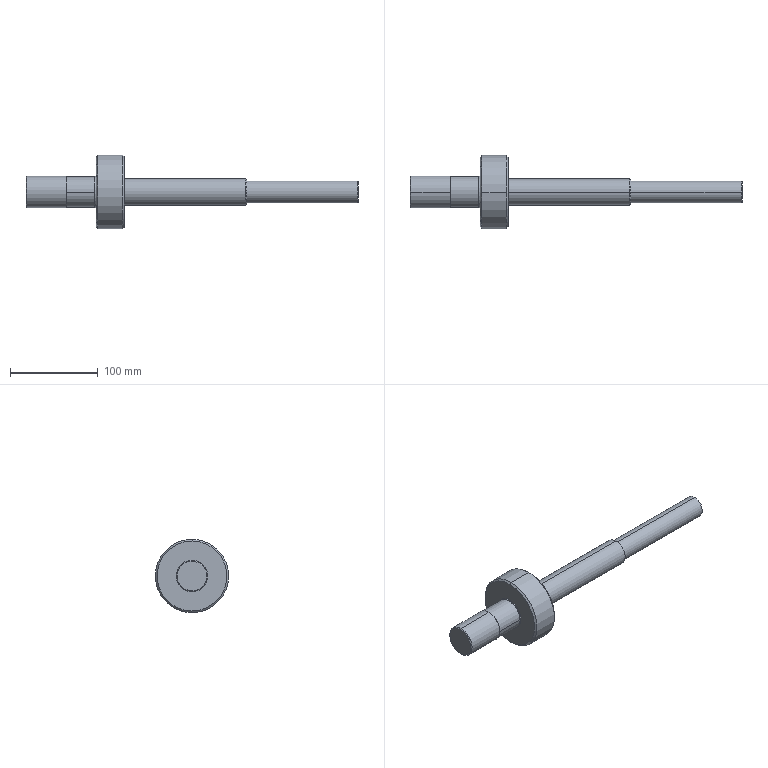Component | SolidWorks | 216InnerTubeAssembly-1_Mandrel1-1 | 1 solid | 29 faces | box 379 x 84 x 84 mm | volume 417048 mm3 | cylinder 12 | cone 10 | plane 7 | commonest cylinder face diameters 36 x4 34.99 x2 25 x2 30 x2 84 x2 | material Alloy Steel
build123d program:
from build123d import *

# Parameters (mm, degrees)
SKETCH1_W = 32.7
SKETCH1_H = 1.005


with BuildPart() as part:
    # Model → Revolve1 (revolve)
    with BuildSketch(Plane.XY, mode=Mode.PRIVATE) as revolve1_sk:
        Polygon((82, 42), (80, 40), (80, 18), (1, 18), (0, 17), (0, 0), (379, 0), (379, 11.5), (378, 12.5), (252, 12.5), (252, 14), (251, 15), (112, 15), (112, 40), (110, 42), align=None)
    revolve(revolve1_sk.sketch.rotate(Axis((388.793, 0, 0), (-1, 0, 0)), 90), axis=Axis((388.793, 0, 0), (-1, 0, 0)))

    # Sketch1 → Cut-Revolve1 (revolve, cut)
    with BuildSketch(Plane.XY, mode=Mode.PRIVATE) as cut_revolve1_sk:
        with Locations((62.371, 17.997)):
            Rectangle(SKETCH1_W, SKETCH1_H)
    revolve(cut_revolve1_sk.sketch.rotate(Axis((41.021, 0, 0), (1, 0, 0)), 270), axis=Axis((41.021, 0, 0), (1, 0, 0)), mode=Mode.SUBTRACT)


solid = part.part

# Placed as in the assembly
solid = solid.moved(Location((714.279, 0, 0), (0, 0, 0)))
STEP:
#1=COLOUR_RGB('',0.7922,0.8196,0.9333);
#2=FILL_AREA_STYLE_COLOUR('',#1);
#3=FILL_AREA_STYLE('',(#2));
#4=SURFACE_STYLE_FILL_AREA(#3);
#5=SURFACE_SIDE_STYLE('',(#4));
#6=SURFACE_STYLE_USAGE(.BOTH.,#5);
#7=PRESENTATION_STYLE_ASSIGNMENT((#6));
#8=CARTESIAN_POINT('',(28.161,0.01272,-0.7085));
#9=VERTEX_POINT('',#8);
#10=CARTESIAN_POINT('',(28.161,-0.01272,0.7085));
#11=VERTEX_POINT('',#10);
#12=CARTESIAN_POINT('',(28.161,-0.,0.));
#13=DIRECTION('',(1.,0.,-0.));
#14=DIRECTION('',(0.,0.01796,-0.9998));
#15=AXIS2_PLACEMENT_3D('',#12,#13,#14);
#16=CIRCLE('',#15,0.7087);
#17=EDGE_CURVE('',#9,#11,#16,.T.);
#18=ORIENTED_EDGE('',*,*,#17,.T.);
#19=CARTESIAN_POINT('',(29.933,-0.01272,0.7085));
#20=VERTEX_POINT('',#19);
#21=CARTESIAN_POINT('',(43.428,-0.01272,0.7085));
#22=DIRECTION('',(1.,0.,-0.));
#23=VECTOR('',#22,39.37);
#24=LINE('',#21,#23);
#25=EDGE_CURVE('',#11,#20,#24,.T.);
#26=ORIENTED_EDGE('',*,*,#25,.T.);
#27=CARTESIAN_POINT('',(29.933,0.01272,-0.7085));
#28=VERTEX_POINT('',#27);
#29=CARTESIAN_POINT('',(29.933,-0.,0.));
#30=DIRECTION('',(-1.,-0.,0.));
#31=DIRECTION('',(0.,0.9998,0.01796));
#32=AXIS2_PLACEMENT_3D('',#29,#30,#31);
#33=CIRCLE('',#32,0.7087);
#34=EDGE_CURVE('',#20,#28,#33,.T.);
#35=ORIENTED_EDGE('',*,*,#34,.T.);
#36=CARTESIAN_POINT('',(43.428,0.01272,-0.7085));
#37=DIRECTION('',(1.,0.,-0.));
#38=VECTOR('',#37,39.37);
#39=LINE('',#36,#38);
#40=EDGE_CURVE('',#9,#28,#39,.T.);
#41=ORIENTED_EDGE('',*,*,#40,.F.);
#42=EDGE_LOOP('',(#18,#26,#35,#41));
#43=FACE_OUTER_BOUND('',#42,.T.);
#44=CARTESIAN_POINT('',(43.428,-0.,0.));
#45=DIRECTION('',(1.,0.,-0.));
#46=DIRECTION('',(0.,0.01796,-0.9998));
#47=AXIS2_PLACEMENT_3D('',#44,#45,#46);
#48=CYLINDRICAL_SURFACE('',#47,0.7087);
#49=ADVANCED_FACE('',(#43),#48,.T.);
#50=CARTESIAN_POINT('',(28.121,0.01202,-0.6692));
#51=VERTEX_POINT('',#50);
#52=CARTESIAN_POINT('',(28.121,-0.01202,0.6692));
#53=VERTEX_POINT('',#52);
#54=CARTESIAN_POINT('',(28.121,-0.,0.));
#55=DIRECTION('',(1.,0.,-0.));
#56=DIRECTION('',(0.,0.01796,-0.9998));
#57=AXIS2_PLACEMENT_3D('',#54,#55,#56);
#58=CIRCLE('',#57,0.6693);
#59=EDGE_CURVE('',#51,#53,#58,.T.);
#60=ORIENTED_EDGE('',*,*,#59,.T.);
#61=CARTESIAN_POINT('',(28.161,-0.01272,0.7085));
#62=DIRECTION('',(0.7071,-0.0127,0.707));
#63=VECTOR('',#62,39.37);
#64=LINE('',#61,#63);
#65=EDGE_CURVE('',#53,#11,#64,.T.);
#66=ORIENTED_EDGE('',*,*,#65,.T.);
#67=ORIENTED_EDGE('',*,*,#17,.F.);
#68=CARTESIAN_POINT('',(28.161,0.01272,-0.7085));
#69=DIRECTION('',(0.7071,0.0127,-0.707));
#70=VECTOR('',#69,39.37);
#71=LINE('',#68,#70);
#72=EDGE_CURVE('',#51,#9,#71,.T.);
#73=ORIENTED_EDGE('',*,*,#72,.F.);
#74=EDGE_LOOP('',(#60,#66,#67,#73));
#75=FACE_OUTER_BOUND('',#74,.T.);
#76=CARTESIAN_POINT('',(28.161,-0.,0.));
#77=DIRECTION('',(1.,0.,-0.));
#78=DIRECTION('',(0.,0.01796,-0.9998));
#79=AXIS2_PLACEMENT_3D('',#76,#77,#78);
#80=CONICAL_SURFACE('',#79,0.7087,0.7854);
#81=ADVANCED_FACE('',(#75),#80,.T.);
#82=CARTESIAN_POINT('',(31.22,-0.6887,-0.01237));
#83=VERTEX_POINT('',#82);
#84=CARTESIAN_POINT('',(31.22,0.6887,0.01237));
#85=VERTEX_POINT('',#84);
#86=CARTESIAN_POINT('',(31.22,-0.,0.));
#87=DIRECTION('',(-1.,-0.,0.));
#88=DIRECTION('',(0.,-0.9998,-0.01796));
#89=AXIS2_PLACEMENT_3D('',#86,#87,#88);
#90=CIRCLE('',#89,0.6888);
#91=EDGE_CURVE('',#83,#85,#90,.T.);
#92=ORIENTED_EDGE('',*,*,#91,.T.);
#93=CARTESIAN_POINT('',(29.933,0.6887,0.01237));
#94=VERTEX_POINT('',#93);
#95=CARTESIAN_POINT('',(29.736,0.6887,0.01237));
#96=DIRECTION('',(-1.,-0.,0.));
#97=VECTOR('',#96,39.37);
#98=LINE('',#95,#97);
#99=EDGE_CURVE('',#85,#94,#98,.T.);
#100=ORIENTED_EDGE('',*,*,#99,.T.);
#101=CARTESIAN_POINT('',(29.933,-0.6887,-0.01237));
#102=VERTEX_POINT('',#101);
#103=CARTESIAN_POINT('',(29.933,-0.,0.));
#104=DIRECTION('',(-1.,-0.,0.));
#105=DIRECTION('',(0.,-0.9998,-0.01796));
#106=AXIS2_PLACEMENT_3D('',#103,#104,#105);
#107=CIRCLE('',#106,0.6888);
#108=EDGE_CURVE('',#102,#94,#107,.T.);
#109=ORIENTED_EDGE('',*,*,#108,.F.);
#110=CARTESIAN_POINT('',(29.736,-0.6887,-0.01237));
#111=DIRECTION('',(-1.,-0.,0.));
#112=VECTOR('',#111,39.37);
#113=LINE('',#110,#112);
#114=EDGE_CURVE('',#83,#102,#113,.T.);
#115=ORIENTED_EDGE('',*,*,#114,.F.);
#116=EDGE_LOOP('',(#92,#100,#109,#115));
#117=FACE_OUTER_BOUND('',#116,.T.);
#118=CARTESIAN_POINT('',(29.736,-0.,0.));
#119=DIRECTION('',(-1.,-0.,0.));
#120=DIRECTION('',(0.,-0.9998,-0.01796));
#121=AXIS2_PLACEMENT_3D('',#118,#119,#120);
#122=CYLINDRICAL_SURFACE('',#121,0.6888);
#123=ADVANCED_FACE('',(#117),#122,.T.);
#124=CARTESIAN_POINT('',(31.271,0.02828,-1.575));
#125=VERTEX_POINT('',#124);
#126=CARTESIAN_POINT('',(31.271,-0.02828,1.575));
#127=VERTEX_POINT('',#126);
#128=CARTESIAN_POINT('',(31.271,-0.,0.));
#129=DIRECTION('',(1.,0.,-0.));
#130=DIRECTION('',(0.,0.01796,-0.9998));
#131=AXIS2_PLACEMENT_3D('',#128,#129,#130);
#132=CIRCLE('',#131,1.575);
#133=EDGE_CURVE('',#125,#127,#132,.T.);
#134=ORIENTED_EDGE('',*,*,#133,.T.);
#135=CARTESIAN_POINT('',(31.35,-0.02969,1.653));
#136=VERTEX_POINT('',#135);
#137=CARTESIAN_POINT('',(31.35,-0.02969,1.653));
#138=DIRECTION('',(0.7071,-0.0127,0.707));
#139=VECTOR('',#138,39.37);
#140=LINE('',#137,#139);
#141=EDGE_CURVE('',#127,#136,#140,.T.);
#142=ORIENTED_EDGE('',*,*,#141,.T.);
#143=CARTESIAN_POINT('',(31.35,0.02969,-1.653));
#144=VERTEX_POINT('',#143);
#145=CARTESIAN_POINT('',(31.35,-0.,0.));
#146=DIRECTION('',(1.,0.,-0.));
#147=DIRECTION('',(0.,0.01796,-0.9998));
#148=AXIS2_PLACEMENT_3D('',#145,#146,#147);
#149=CIRCLE('',#148,1.654);
#150=EDGE_CURVE('',#144,#136,#149,.T.);
#151=ORIENTED_EDGE('',*,*,#150,.F.);
#152=CARTESIAN_POINT('',(31.35,0.02969,-1.653));
#153=DIRECTION('',(0.7071,0.0127,-0.707));
#154=VECTOR('',#153,39.37);
#155=LINE('',#152,#154);
#156=EDGE_CURVE('',#125,#144,#155,.T.);
#157=ORIENTED_EDGE('',*,*,#156,.F.);
#158=EDGE_LOOP('',(#134,#142,#151,#157));
#159=FACE_OUTER_BOUND('',#158,.T.);
#160=CARTESIAN_POINT('',(31.35,-0.,0.));
#161=DIRECTION('',(1.,0.,-0.));
#162=DIRECTION('',(0.,0.01796,-0.9998));
#163=AXIS2_PLACEMENT_3D('',#160,#161,#162);
#164=CONICAL_SURFACE('',#163,1.654,0.7854);
#165=ADVANCED_FACE('',(#159),#164,.T.);
#166=CARTESIAN_POINT('',(43.042,0.00813,-0.4527));
#167=VERTEX_POINT('',#166);
#168=CARTESIAN_POINT('',(43.042,-0.00813,0.4527));
#169=VERTEX_POINT('',#168);
#170=CARTESIAN_POINT('',(43.042,-0.,0.));
#171=DIRECTION('',(1.,0.,-0.));
#172=DIRECTION('',(0.,0.01796,-0.9998));
#173=AXIS2_PLACEMENT_3D('',#170,#171,#172);
#174=CIRCLE('',#173,0.4528);
#175=EDGE_CURVE('',#167,#169,#174,.T.);
#176=ORIENTED_EDGE('',*,*,#175,.F.);
#177=CARTESIAN_POINT('',(43.003,0.008837,-0.492));
#178=VERTEX_POINT('',#177);
#179=CARTESIAN_POINT('',(43.042,0.00813,-0.4527));
#180=DIRECTION('',(-0.7071,0.0127,-0.707));
#181=VECTOR('',#180,39.37);
#182=LINE('',#179,#181);
#183=EDGE_CURVE('',#167,#178,#182,.T.);
#184=ORIENTED_EDGE('',*,*,#183,.T.);
#185=CARTESIAN_POINT('',(43.003,-0.008837,0.492));
#186=VERTEX_POINT('',#185);
#187=CARTESIAN_POINT('',(43.003,-0.,0.));
#188=DIRECTION('',(1.,0.,-0.));
#189=DIRECTION('',(0.,0.01796,-0.9998));
#190=AXIS2_PLACEMENT_3D('',#187,#188,#189);
#191=CIRCLE('',#190,0.4921);
#192=EDGE_CURVE('',#178,#186,#191,.T.);
#193=ORIENTED_EDGE('',*,*,#192,.T.);
#194=CARTESIAN_POINT('',(43.042,-0.00813,0.4527));
#195=DIRECTION('',(-0.7071,-0.0127,0.707));
#196=VECTOR('',#195,39.37);
#197=LINE('',#194,#196);
#198=EDGE_CURVE('',#169,#186,#197,.T.);
#199=ORIENTED_EDGE('',*,*,#198,.F.);
#200=EDGE_LOOP('',(#176,#184,#193,#199));
#201=FACE_OUTER_BOUND('',#200,.T.);
#202=CARTESIAN_POINT('',(43.042,-0.,0.));
#203=DIRECTION('',(-1.,-0.,0.));
#204=DIRECTION('',(0.,-0.01796,0.9998));
#205=AXIS2_PLACEMENT_3D('',#202,#203,#204);
#206=CONICAL_SURFACE('',#205,0.4528,0.7854);
#207=ADVANCED_FACE('',(#201),#206,.T.);
#208=CARTESIAN_POINT('',(38.042,0.008837,-0.492));
#209=VERTEX_POINT('',#208);
#210=CARTESIAN_POINT('',(38.042,-0.008837,0.492));
#211=VERTEX_POINT('',#210);
#212=CARTESIAN_POINT('',(38.042,-0.,0.));
#213=DIRECTION('',(1.,0.,-0.));
#214=DIRECTION('',(0.,0.01796,-0.9998));
#215=AXIS2_PLACEMENT_3D('',#212,#213,#214);
#216=CIRCLE('',#215,0.4921);
#217=EDGE_CURVE('',#209,#211,#216,.T.);
#218=ORIENTED_EDGE('',*,*,#217,.T.);
#219=CARTESIAN_POINT('',(43.428,-0.008837,0.492));
#220=DIRECTION('',(1.,0.,-0.));
#221=VECTOR('',#220,39.37);
#222=LINE('',#219,#221);
#223=EDGE_CURVE('',#211,#186,#222,.T.);
#224=ORIENTED_EDGE('',*,*,#223,.T.);
#225=ORIENTED_EDGE('',*,*,#192,.F.);
#226=CARTESIAN_POINT('',(43.428,0.008837,-0.492));
#227=DIRECTION('',(1.,0.,-0.));
#228=VECTOR('',#227,39.37);
#229=LINE('',#226,#228);
#230=EDGE_CURVE('',#209,#178,#229,.T.);
#231=ORIENTED_EDGE('',*,*,#230,.F.);
#232=EDGE_LOOP('',(#218,#224,#225,#231));
#233=FACE_OUTER_BOUND('',#232,.T.);
#234=CARTESIAN_POINT('',(43.428,-0.,0.));
#235=DIRECTION('',(1.,0.,-0.));
#236=DIRECTION('',(0.,0.01796,-0.9998));
#237=AXIS2_PLACEMENT_3D('',#234,#235,#236);
#238=CYLINDRICAL_SURFACE('',#237,0.4921);
#239=ADVANCED_FACE('',(#233),#238,.T.);
#240=CARTESIAN_POINT('',(38.042,0.009897,-0.5511));
#241=VERTEX_POINT('',#240);
#242=CARTESIAN_POINT('',(38.042,-0.009897,0.5511));
#243=VERTEX_POINT('',#242);
#244=CARTESIAN_POINT('',(38.042,-0.,0.));
#245=DIRECTION('',(1.,0.,-0.));
#246=DIRECTION('',(0.,0.01796,-0.9998));
#247=AXIS2_PLACEMENT_3D('',#244,#245,#246);
#248=CIRCLE('',#247,0.5512);
#249=EDGE_CURVE('',#241,#243,#248,.T.);
#250=ORIENTED_EDGE('',*,*,#249,.F.);
#251=CARTESIAN_POINT('',(38.003,0.0106,-0.5905));
#252=VERTEX_POINT('',#251);
#253=CARTESIAN_POINT('',(38.042,0.009897,-0.5511));
#254=DIRECTION('',(-0.7071,0.0127,-0.707));
#255=VECTOR('',#254,39.37);
#256=LINE('',#253,#255);
#257=EDGE_CURVE('',#241,#252,#256,.T.);
#258=ORIENTED_EDGE('',*,*,#257,.T.);
#259=CARTESIAN_POINT('',(38.003,-0.0106,0.5905));
#260=VERTEX_POINT('',#259);
#261=CARTESIAN_POINT('',(38.003,-0.,0.));
#262=DIRECTION('',(1.,0.,-0.));
#263=DIRECTION('',(0.,0.01796,-0.9998));
#264=AXIS2_PLACEMENT_3D('',#261,#262,#263);
#265=CIRCLE('',#264,0.5906);
#266=EDGE_CURVE('',#252,#260,#265,.T.);
#267=ORIENTED_EDGE('',*,*,#266,.T.);
#268=CARTESIAN_POINT('',(38.042,-0.009897,0.5511));
#269=DIRECTION('',(-0.7071,-0.0127,0.707));
#270=VECTOR('',#269,39.37);
#271=LINE('',#268,#270);
#272=EDGE_CURVE('',#243,#260,#271,.T.);
#273=ORIENTED_EDGE('',*,*,#272,.F.);
#274=EDGE_LOOP('',(#250,#258,#267,#273));
#275=FACE_OUTER_BOUND('',#274,.T.);
#276=CARTESIAN_POINT('',(38.042,-0.,0.));
#277=DIRECTION('',(-1.,-0.,0.));
#278=DIRECTION('',(0.,-0.01796,0.9998));
#279=AXIS2_PLACEMENT_3D('',#276,#277,#278);
#280=CONICAL_SURFACE('',#279,0.5512,0.7854);
#281=ADVANCED_FACE('',(#275),#280,.T.);
#282=CARTESIAN_POINT('',(32.531,0.0106,-0.5905));
#283=VERTEX_POINT('',#282);
#284=CARTESIAN_POINT('',(32.531,-0.0106,0.5905));
#285=VERTEX_POINT('',#284);
#286=CARTESIAN_POINT('',(32.531,-0.,0.));
#287=DIRECTION('',(1.,0.,-0.));
#288=DIRECTION('',(0.,0.01796,-0.9998));
#289=AXIS2_PLACEMENT_3D('',#286,#287,#288);
#290=CIRCLE('',#289,0.5906);
#291=EDGE_CURVE('',#283,#285,#290,.T.);
#292=ORIENTED_EDGE('',*,*,#291,.T.);
#293=CARTESIAN_POINT('',(43.428,-0.0106,0.5905));
#294=DIRECTION('',(1.,0.,-0.));
#295=VECTOR('',#294,39.37);
#296=LINE('',#293,#295);
#297=EDGE_CURVE('',#285,#260,#296,.T.);
#298=ORIENTED_EDGE('',*,*,#297,.T.);
#299=ORIENTED_EDGE('',*,*,#266,.F.);
#300=CARTESIAN_POINT('',(43.428,0.0106,-0.5905));
#301=DIRECTION('',(1.,0.,-0.));
#302=VECTOR('',#301,39.37);
#303=LINE('',#300,#302);
#304=EDGE_CURVE('',#283,#252,#303,.T.);
#305=ORIENTED_EDGE('',*,*,#304,.F.);
#306=EDGE_LOOP('',(#292,#298,#299,#305));
#307=FACE_OUTER_BOUND('',#306,.T.);
#308=CARTESIAN_POINT('',(43.428,-0.,0.));
#309=DIRECTION('',(1.,0.,-0.));
#310=DIRECTION('',(0.,0.01796,-0.9998));
#311=AXIS2_PLACEMENT_3D('',#308,#309,#310);
#312=CYLINDRICAL_SURFACE('',#311,0.5906);
#313=ADVANCED_FACE('',(#307),#312,.T.);
#314=CARTESIAN_POINT('',(32.531,0.02828,-1.575));
#315=VERTEX_POINT('',#314);
#316=CARTESIAN_POINT('',(32.531,-0.02828,1.575));
#317=VERTEX_POINT('',#316);
#318=CARTESIAN_POINT('',(32.531,-0.,0.));
#319=DIRECTION('',(1.,0.,-0.));
#320=DIRECTION('',(0.,0.01796,-0.9998));
#321=AXIS2_PLACEMENT_3D('',#318,#319,#320);
#322=CIRCLE('',#321,1.575);
#323=EDGE_CURVE('',#315,#317,#322,.T.);
#324=ORIENTED_EDGE('',*,*,#323,.F.);
#325=CARTESIAN_POINT('',(32.452,0.02969,-1.653));
#326=VERTEX_POINT('',#325);
#327=CARTESIAN_POINT('',(32.531,0.02828,-1.575));
#328=DIRECTION('',(-0.7071,0.0127,-0.707));
#329=VECTOR('',#328,39.37);
#330=LINE('',#327,#329);
#331=EDGE_CURVE('',#315,#326,#330,.T.);
#332=ORIENTED_EDGE('',*,*,#331,.T.);
#333=CARTESIAN_POINT('',(32.452,-0.02969,1.653));
#334=VERTEX_POINT('',#333);
#335=CARTESIAN_POINT('',(32.452,-0.,0.));
#336=DIRECTION('',(1.,0.,-0.));
#337=DIRECTION('',(0.,0.01796,-0.9998));
#338=AXIS2_PLACEMENT_3D('',#335,#336,#337);
#339=CIRCLE('',#338,1.654);
#340=EDGE_CURVE('',#326,#334,#339,.T.);
#341=ORIENTED_EDGE('',*,*,#340,.T.);
#342=CARTESIAN_POINT('',(32.531,-0.02828,1.575));
#343=DIRECTION('',(-0.7071,-0.0127,0.707));
#344=VECTOR('',#343,39.37);
#345=LINE('',#342,#344);
#346=EDGE_CURVE('',#317,#334,#345,.T.);
#347=ORIENTED_EDGE('',*,*,#346,.F.);
#348=EDGE_LOOP('',(#324,#332,#341,#347));
#349=FACE_OUTER_BOUND('',#348,.T.);
#350=CARTESIAN_POINT('',(32.531,-0.,0.));
#351=DIRECTION('',(-1.,-0.,0.));
#352=DIRECTION('',(0.,-0.01796,0.9998));
#353=AXIS2_PLACEMENT_3D('',#350,#351,#352);
#354=CONICAL_SURFACE('',#353,1.575,0.7854);
#355=ADVANCED_FACE('',(#349),#354,.T.);
#356=ORIENTED_EDGE('',*,*,#150,.T.);
#357=CARTESIAN_POINT('',(43.428,-0.02969,1.653));
#358=DIRECTION('',(1.,0.,-0.));
#359=VECTOR('',#358,39.37);
#360=LINE('',#357,#359);
#361=EDGE_CURVE('',#136,#334,#360,.T.);
#362=ORIENTED_EDGE('',*,*,#361,.T.);
#363=ORIENTED_EDGE('',*,*,#340,.F.);
#364=CARTESIAN_POINT('',(43.428,0.02969,-1.653));
#365=DIRECTION('',(1.,0.,-0.));
#366=VECTOR('',#365,39.37);
#367=LINE('',#364,#366);
#368=EDGE_CURVE('',#144,#326,#367,.T.);
#369=ORIENTED_EDGE('',*,*,#368,.F.);
#370=EDGE_LOOP('',(#356,#362,#363,#369));
#371=FACE_OUTER_BOUND('',#370,.T.);
#372=CARTESIAN_POINT('',(43.428,-0.,0.));
#373=DIRECTION('',(1.,0.,-0.));
#374=DIRECTION('',(0.,0.01796,-0.9998));
#375=AXIS2_PLACEMENT_3D('',#372,#373,#374);
#376=CYLINDRICAL_SURFACE('',#375,1.654);
#377=ADVANCED_FACE('',(#371),#376,.T.);
#378=CARTESIAN_POINT('',(31.22,0.01272,-0.7085));
#379=VERTEX_POINT('',#378);
#380=CARTESIAN_POINT('',(31.22,-0.01272,0.7085));
#381=VERTEX_POINT('',#380);
#382=CARTESIAN_POINT('',(31.22,-0.,0.));
#383=DIRECTION('',(1.,0.,-0.));
#384=DIRECTION('',(0.,-0.9998,-0.01796));
#385=AXIS2_PLACEMENT_3D('',#382,#383,#384);
#386=CIRCLE('',#385,0.7087);
#387=EDGE_CURVE('',#379,#381,#386,.T.);
#388=ORIENTED_EDGE('',*,*,#387,.T.);
#389=CARTESIAN_POINT('',(31.271,-0.01272,0.7085));
#390=VERTEX_POINT('',#389);
#391=CARTESIAN_POINT('',(43.428,-0.01272,0.7085));
#392=DIRECTION('',(1.,0.,-0.));
#393=VECTOR('',#392,39.37);
#394=LINE('',#391,#393);
#395=EDGE_CURVE('',#381,#390,#394,.T.);
#396=ORIENTED_EDGE('',*,*,#395,.T.);
#397=CARTESIAN_POINT('',(31.271,0.01272,-0.7085));
#398=VERTEX_POINT('',#397);
#399=CARTESIAN_POINT('',(31.271,-0.,0.));
#400=DIRECTION('',(1.,0.,-0.));
#401=DIRECTION('',(0.,0.01796,-0.9998));
#402=AXIS2_PLACEMENT_3D('',#399,#400,#401);
#403=CIRCLE('',#402,0.7087);
#404=EDGE_CURVE('',#398,#390,#403,.T.);
#405=ORIENTED_EDGE('',*,*,#404,.F.);
#406=CARTESIAN_POINT('',(43.428,0.01272,-0.7085));
#407=DIRECTION('',(1.,0.,-0.));
#408=VECTOR('',#407,39.37);
#409=LINE('',#406,#408);
#410=EDGE_CURVE('',#379,#398,#409,.T.);
#411=ORIENTED_EDGE('',*,*,#410,.F.);
#412=EDGE_LOOP('',(#388,#396,#405,#411));
#413=FACE_OUTER_BOUND('',#412,.T.);
#414=CARTESIAN_POINT('',(43.428,-0.,0.));
#415=DIRECTION('',(1.,0.,-0.));
#416=DIRECTION('',(0.,0.01796,-0.9998));
#417=AXIS2_PLACEMENT_3D('',#414,#415,#416);
#418=CYLINDRICAL_SURFACE('',#417,0.7087);
#419=ADVANCED_FACE('',(#413),#418,.T.);
#420=ORIENTED_EDGE('',*,*,#395,.F.);
#421=CARTESIAN_POINT('',(31.22,-0.,0.));
#422=DIRECTION('',(1.,0.,-0.));
#423=DIRECTION('',(0.,-0.9998,-0.01796));
#424=AXIS2_PLACEMENT_3D('',#421,#422,#423);
#425=CIRCLE('',#424,0.7087);
#426=EDGE_CURVE('',#381,#379,#425,.T.);
#427=ORIENTED_EDGE('',*,*,#426,.T.);
#428=ORIENTED_EDGE('',*,*,#410,.T.);
#429=CARTESIAN_POINT('',(31.271,-0.,0.));
#430=DIRECTION('',(1.,0.,-0.));
#431=DIRECTION('',(0.,0.01796,-0.9998));
#432=AXIS2_PLACEMENT_3D('',#429,#430,#431);
#433=CIRCLE('',#432,0.7087);
#434=EDGE_CURVE('',#390,#398,#433,.T.);
#435=ORIENTED_EDGE('',*,*,#434,.F.);
#436=EDGE_LOOP('',(#420,#427,#428,#435));
#437=FACE_OUTER_BOUND('',#436,.T.);
#438=CARTESIAN_POINT('',(43.428,-0.,0.));
#439=DIRECTION('',(1.,0.,-0.));
#440=DIRECTION('',(0.,0.01796,-0.9998));
#441=AXIS2_PLACEMENT_3D('',#438,#439,#440);
#442=CYLINDRICAL_SURFACE('',#441,0.7087);
#443=ADVANCED_FACE('',(#437),#442,.T.);
#444=ORIENTED_EDGE('',*,*,#361,.F.);
#445=CARTESIAN_POINT('',(31.35,-0.,0.));
#446=DIRECTION('',(1.,0.,-0.));
#447=DIRECTION('',(0.,0.01796,-0.9998));
#448=AXIS2_PLACEMENT_3D('',#445,#446,#447);
#449=CIRCLE('',#448,1.654);
#450=EDGE_CURVE('',#136,#144,#449,.T.);
#451=ORIENTED_EDGE('',*,*,#450,.T.);
#452=ORIENTED_EDGE('',*,*,#368,.T.);
#453=CARTESIAN_POINT('',(32.452,-0.,0.));
#454=DIRECTION('',(1.,0.,-0.));
#455=DIRECTION('',(0.,0.01796,-0.9998));
#456=AXIS2_PLACEMENT_3D('',#453,#454,#455);
#457=CIRCLE('',#456,1.654);
#458=EDGE_CURVE('',#334,#326,#457,.T.);
#459=ORIENTED_EDGE('',*,*,#458,.F.);
#460=EDGE_LOOP('',(#444,#451,#452,#459));
#461=FACE_OUTER_BOUND('',#460,.T.);
#462=CARTESIAN_POINT('',(43.428,-0.,0.));
#463=DIRECTION('',(1.,0.,-0.));
#464=DIRECTION('',(0.,0.01796,-0.9998));
#465=AXIS2_PLACEMENT_3D('',#462,#463,#464);
#466=CYLINDRICAL_SURFACE('',#465,1.654);
#467=ADVANCED_FACE('',(#461),#466,.T.);
#468=ORIENTED_EDGE('',*,*,#331,.F.);
#469=CARTESIAN_POINT('',(32.531,-0.,0.));
#470=DIRECTION('',(1.,0.,-0.));
#471=DIRECTION('',(0.,0.01796,-0.9998));
#472=AXIS2_PLACEMENT_3D('',#469,#470,#471);
#473=CIRCLE('',#472,1.575);
#474=EDGE_CURVE('',#317,#315,#473,.T.);
#475=ORIENTED_EDGE('',*,*,#474,.F.);
#476=ORIENTED_EDGE('',*,*,#346,.T.);
#477=ORIENTED_EDGE('',*,*,#458,.T.);
#478=EDGE_LOOP('',(#468,#475,#476,#477));
#479=FACE_OUTER_BOUND('',#478,.T.);
#480=CARTESIAN_POINT('',(32.531,-0.,0.));
#481=DIRECTION('',(-1.,-0.,0.));
#482=DIRECTION('',(0.,-0.01796,0.9998));
#483=AXIS2_PLACEMENT_3D('',#480,#481,#482);
#484=CONICAL_SURFACE('',#483,1.575,0.7854);
#485=ADVANCED_FACE('',(#479),#484,.T.);
#486=ORIENTED_EDGE('',*,*,#474,.T.);
#487=ORIENTED_EDGE('',*,*,#323,.T.);
#488=EDGE_LOOP('',(#486,#487));
#489=FACE_OUTER_BOUND('',#488,.T.);
#490=ORIENTED_EDGE('',*,*,#291,.F.);
#491=CARTESIAN_POINT('',(32.531,-0.,0.));
#492=DIRECTION('',(1.,0.,-0.));
#493=DIRECTION('',(0.,0.01796,-0.9998));
#494=AXIS2_PLACEMENT_3D('',#491,#492,#493);
#495=CIRCLE('',#494,0.5906);
#496=EDGE_CURVE('',#285,#283,#495,.T.);
#497=ORIENTED_EDGE('',*,*,#496,.F.);
#498=EDGE_LOOP('',(#490,#497));
#499=FACE_BOUND('',#498,.T.);
#500=CARTESIAN_POINT('',(32.531,0.5905,0.0106));
#501=DIRECTION('',(1.,0.,-0.));
#502=DIRECTION('',(-0.,0.01796,-0.9998));
#503=AXIS2_PLACEMENT_3D('',#500,#501,#502);
#504=PLANE('',#503);
#505=ADVANCED_FACE('',(#489,#499),#504,.T.);
#506=ORIENTED_EDGE('',*,*,#297,.F.);
#507=ORIENTED_EDGE('',*,*,#496,.T.);
#508=ORIENTED_EDGE('',*,*,#304,.T.);
#509=CARTESIAN_POINT('',(38.003,-0.,0.));
#510=DIRECTION('',(1.,0.,-0.));
#511=DIRECTION('',(0.,0.01796,-0.9998));
#512=AXIS2_PLACEMENT_3D('',#509,#510,#511);
#513=CIRCLE('',#512,0.5906);
#514=EDGE_CURVE('',#260,#252,#513,.T.);
#515=ORIENTED_EDGE('',*,*,#514,.F.);
#516=EDGE_LOOP('',(#506,#507,#508,#515));
#517=FACE_OUTER_BOUND('',#516,.T.);
#518=CARTESIAN_POINT('',(43.428,-0.,0.));
#519=DIRECTION('',(1.,0.,-0.));
#520=DIRECTION('',(0.,0.01796,-0.9998));
#521=AXIS2_PLACEMENT_3D('',#518,#519,#520);
#522=CYLINDRICAL_SURFACE('',#521,0.5906);
#523=ADVANCED_FACE('',(#517),#522,.T.);
#524=ORIENTED_EDGE('',*,*,#257,.F.);
#525=CARTESIAN_POINT('',(38.042,-0.,0.));
#526=DIRECTION('',(1.,0.,-0.));
#527=DIRECTION('',(0.,0.01796,-0.9998));
#528=AXIS2_PLACEMENT_3D('',#525,#526,#527);
#529=CIRCLE('',#528,0.5512);
#530=EDGE_CURVE('',#243,#241,#529,.T.);
#531=ORIENTED_EDGE('',*,*,#530,.F.);
#532=ORIENTED_EDGE('',*,*,#272,.T.);
#533=ORIENTED_EDGE('',*,*,#514,.T.);
#534=EDGE_LOOP('',(#524,#531,#532,#533));
#535=FACE_OUTER_BOUND('',#534,.T.);
#536=CARTESIAN_POINT('',(38.042,-0.,0.));
#537=DIRECTION('',(-1.,-0.,0.));
#538=DIRECTION('',(0.,-0.01796,0.9998));
#539=AXIS2_PLACEMENT_3D('',#536,#537,#538);
#540=CONICAL_SURFACE('',#539,0.5512,0.7854);
#541=ADVANCED_FACE('',(#535),#540,.T.);
#542=ORIENTED_EDGE('',*,*,#530,.T.);
#543=ORIENTED_EDGE('',*,*,#249,.T.);
#544=EDGE_LOOP('',(#542,#543));
#545=FACE_OUTER_BOUND('',#544,.T.);
#546=ORIENTED_EDGE('',*,*,#217,.F.);
#547=CARTESIAN_POINT('',(38.042,-0.,0.));
#548=DIRECTION('',(1.,0.,-0.));
#549=DIRECTION('',(0.,0.01796,-0.9998));
#550=AXIS2_PLACEMENT_3D('',#547,#548,#549);
#551=CIRCLE('',#550,0.4921);
#552=EDGE_CURVE('',#211,#209,#551,.T.);
#553=ORIENTED_EDGE('',*,*,#552,.F.);
#554=EDGE_LOOP('',(#546,#553));
#555=FACE_BOUND('',#554,.T.);
#556=CARTESIAN_POINT('',(38.042,0.492,0.008837));
#557=DIRECTION('',(1.,0.,-0.));
#558=DIRECTION('',(-0.,0.01796,-0.9998));
#559=AXIS2_PLACEMENT_3D('',#556,#557,#558);
#560=PLANE('',#559);
#561=ADVANCED_FACE('',(#545,#555),#560,.T.);
#562=ORIENTED_EDGE('',*,*,#223,.F.);
#563=ORIENTED_EDGE('',*,*,#552,.T.);
#564=ORIENTED_EDGE('',*,*,#230,.T.);
#565=CARTESIAN_POINT('',(43.003,-0.,0.));
#566=DIRECTION('',(1.,0.,-0.));
#567=DIRECTION('',(0.,0.01796,-0.9998));
#568=AXIS2_PLACEMENT_3D('',#565,#566,#567);
#569=CIRCLE('',#568,0.4921);
#570=EDGE_CURVE('',#186,#178,#569,.T.);
#571=ORIENTED_EDGE('',*,*,#570,.F.);
#572=EDGE_LOOP('',(#562,#563,#564,#571));
#573=FACE_OUTER_BOUND('',#572,.T.);
#574=CARTESIAN_POINT('',(43.428,-0.,0.));
#575=DIRECTION('',(1.,0.,-0.));
#576=DIRECTION('',(0.,0.01796,-0.9998));
#577=AXIS2_PLACEMENT_3D('',#574,#575,#576);
#578=CYLINDRICAL_SURFACE('',#577,0.4921);
#579=ADVANCED_FACE('',(#573),#578,.T.);
#580=ORIENTED_EDGE('',*,*,#183,.F.);
#581=CARTESIAN_POINT('',(43.042,-0.,0.));
#582=DIRECTION('',(1.,0.,-0.));
#583=DIRECTION('',(0.,0.01796,-0.9998));
#584=AXIS2_PLACEMENT_3D('',#581,#582,#583);
#585=CIRCLE('',#584,0.4528);
#586=EDGE_CURVE('',#169,#167,#585,.T.);
#587=ORIENTED_EDGE('',*,*,#586,.F.);
#588=ORIENTED_EDGE('',*,*,#198,.T.);
#589=ORIENTED_EDGE('',*,*,#570,.T.);
#590=EDGE_LOOP('',(#580,#587,#588,#589));
#591=FACE_OUTER_BOUND('',#590,.T.);
#592=CARTESIAN_POINT('',(43.042,-0.,0.));
#593=DIRECTION('',(-1.,-0.,0.));
#594=DIRECTION('',(0.,-0.01796,0.9998));
#595=AXIS2_PLACEMENT_3D('',#592,#593,#594);
#596=CONICAL_SURFACE('',#595,0.4528,0.7854);
#597=ADVANCED_FACE('',(#591),#596,.T.);
#598=ORIENTED_EDGE('',*,*,#586,.T.);
#599=ORIENTED_EDGE('',*,*,#175,.T.);
#600=EDGE_LOOP('',(#598,#599));
#601=FACE_OUTER_BOUND('',#600,.T.);
#602=CARTESIAN_POINT('',(43.042,-0.,0.));
#603=DIRECTION('',(1.,0.,-0.));
#604=DIRECTION('',(-0.,0.01796,-0.9998));
#605=AXIS2_PLACEMENT_3D('',#602,#603,#604);
#606=PLANE('',#605);
#607=ADVANCED_FACE('',(#601),#606,.T.);
#608=ORIENTED_EDGE('',*,*,#404,.T.);
#609=ORIENTED_EDGE('',*,*,#434,.T.);
#610=EDGE_LOOP('',(#608,#609));
#611=FACE_BOUND('',#610,.T.);
#612=ORIENTED_EDGE('',*,*,#133,.F.);
#613=CARTESIAN_POINT('',(31.271,-0.,0.));
#614=DIRECTION('',(1.,0.,-0.));
#615=DIRECTION('',(0.,0.01796,-0.9998));
#616=AXIS2_PLACEMENT_3D('',#613,#614,#615);
#617=CIRCLE('',#616,1.575);
#618=EDGE_CURVE('',#127,#125,#617,.T.);
#619=ORIENTED_EDGE('',*,*,#618,.F.);
#620=EDGE_LOOP('',(#612,#619));
#621=FACE_OUTER_BOUND('',#620,.T.);
#622=CARTESIAN_POINT('',(31.271,0.7085,0.01272));
#623=DIRECTION('',(-1.,-0.,0.));
#624=DIRECTION('',(0.,-0.01796,0.9998));
#625=AXIS2_PLACEMENT_3D('',#622,#623,#624);
#626=PLANE('',#625);
#627=ADVANCED_FACE('',(#611,#621),#626,.T.);
#628=ORIENTED_EDGE('',*,*,#141,.F.);
#629=ORIENTED_EDGE('',*,*,#618,.T.);
#630=ORIENTED_EDGE('',*,*,#156,.T.);
#631=ORIENTED_EDGE('',*,*,#450,.F.);
#632=EDGE_LOOP('',(#628,#629,#630,#631));
#633=FACE_OUTER_BOUND('',#632,.T.);
#634=CARTESIAN_POINT('',(31.35,-0.,0.));
#635=DIRECTION('',(1.,0.,-0.));
#636=DIRECTION('',(0.,0.01796,-0.9998));
#637=AXIS2_PLACEMENT_3D('',#634,#635,#636);
#638=CONICAL_SURFACE('',#637,1.654,0.7854);
#639=ADVANCED_FACE('',(#633),#638,.T.);
#640=ORIENTED_EDGE('',*,*,#99,.F.);
#641=CARTESIAN_POINT('',(31.22,-0.,0.));
#642=DIRECTION('',(-1.,-0.,0.));
#643=DIRECTION('',(0.,-0.9998,-0.01796));
#644=AXIS2_PLACEMENT_3D('',#641,#642,#643);
#645=CIRCLE('',#644,0.6888);
#646=EDGE_CURVE('',#85,#83,#645,.T.);
#647=ORIENTED_EDGE('',*,*,#646,.T.);
#648=ORIENTED_EDGE('',*,*,#114,.T.);
#649=CARTESIAN_POINT('',(29.933,-0.,0.));
#650=DIRECTION('',(-1.,-0.,0.));
#651=DIRECTION('',(0.,-0.9998,-0.01796));
#652=AXIS2_PLACEMENT_3D('',#649,#650,#651);
#653=CIRCLE('',#652,0.6888);
#654=EDGE_CURVE('',#94,#102,#653,.T.);
#655=ORIENTED_EDGE('',*,*,#654,.F.);
#656=EDGE_LOOP('',(#640,#647,#648,#655));
#657=FACE_OUTER_BOUND('',#656,.T.);
#658=CARTESIAN_POINT('',(29.736,-0.,0.));
#659=DIRECTION('',(-1.,-0.,0.));
#660=DIRECTION('',(0.,-0.9998,-0.01796));
#661=AXIS2_PLACEMENT_3D('',#658,#659,#660);
#662=CYLINDRICAL_SURFACE('',#661,0.6888);
#663=ADVANCED_FACE('',(#657),#662,.T.);
#664=CARTESIAN_POINT('',(29.933,-0.,0.));
#665=DIRECTION('',(-1.,-0.,0.));
#666=DIRECTION('',(0.,0.9998,0.01796));
#667=AXIS2_PLACEMENT_3D('',#664,#665,#666);
#668=CIRCLE('',#667,0.7087);
#669=EDGE_CURVE('',#28,#20,#668,.T.);
#670=ORIENTED_EDGE('',*,*,#669,.F.);
#671=ORIENTED_EDGE('',*,*,#34,.F.);
#672=EDGE_LOOP('',(#670,#671));
#673=FACE_OUTER_BOUND('',#672,.T.);
#674=ORIENTED_EDGE('',*,*,#108,.T.);
#675=ORIENTED_EDGE('',*,*,#654,.T.);
#676=EDGE_LOOP('',(#674,#675));
#677=FACE_BOUND('',#676,.T.);
#678=CARTESIAN_POINT('',(29.933,0.6887,0.01237));
#679=DIRECTION('',(1.,0.,-0.));
#680=DIRECTION('',(0.,0.9998,0.01796));
#681=AXIS2_PLACEMENT_3D('',#678,#679,#680);
#682=PLANE('',#681);
#683=ADVANCED_FACE('',(#673,#677),#682,.T.);
#684=ORIENTED_EDGE('',*,*,#387,.F.);
#685=ORIENTED_EDGE('',*,*,#426,.F.);
#686=EDGE_LOOP('',(#684,#685));
#687=FACE_OUTER_BOUND('',#686,.T.);
#688=ORIENTED_EDGE('',*,*,#91,.F.);
#689=ORIENTED_EDGE('',*,*,#646,.F.);
#690=EDGE_LOOP('',(#688,#689));
#691=FACE_BOUND('',#690,.T.);
#692=CARTESIAN_POINT('',(31.22,0.7282,0.01308));
#693=DIRECTION('',(-1.,-0.,0.));
#694=DIRECTION('',(-0.,-0.9998,-0.01796));
#695=AXIS2_PLACEMENT_3D('',#692,#693,#694);
#696=PLANE('',#695);
#697=ADVANCED_FACE('',(#687,#691),#696,.T.);
#698=ORIENTED_EDGE('',*,*,#59,.F.);
#699=CARTESIAN_POINT('',(28.121,-0.,0.));
#700=DIRECTION('',(1.,0.,-0.));
#701=DIRECTION('',(0.,0.01796,-0.9998));
#702=AXIS2_PLACEMENT_3D('',#699,#700,#701);
#703=CIRCLE('',#702,0.6693);
#704=EDGE_CURVE('',#53,#51,#703,.T.);
#705=ORIENTED_EDGE('',*,*,#704,.F.);
#706=EDGE_LOOP('',(#698,#705));
#707=FACE_OUTER_BOUND('',#706,.T.);
#708=CARTESIAN_POINT('',(28.121,-0.,0.));
#709=DIRECTION('',(-1.,-0.,0.));
#710=DIRECTION('',(0.,-0.01796,0.9998));
#711=AXIS2_PLACEMENT_3D('',#708,#709,#710);
#712=PLANE('',#711);
#713=ADVANCED_FACE('',(#707),#712,.T.);
#714=ORIENTED_EDGE('',*,*,#65,.F.);
#715=ORIENTED_EDGE('',*,*,#704,.T.);
#716=ORIENTED_EDGE('',*,*,#72,.T.);
#717=CARTESIAN_POINT('',(28.161,-0.,0.));
#718=DIRECTION('',(1.,0.,-0.));
#719=DIRECTION('',(0.,0.01796,-0.9998));
#720=AXIS2_PLACEMENT_3D('',#717,#718,#719);
#721=CIRCLE('',#720,0.7087);
#722=EDGE_CURVE('',#11,#9,#721,.T.);
#723=ORIENTED_EDGE('',*,*,#722,.F.);
#724=EDGE_LOOP('',(#714,#715,#716,#723));
#725=FACE_OUTER_BOUND('',#724,.T.);
#726=CARTESIAN_POINT('',(28.161,-0.,0.));
#727=DIRECTION('',(1.,0.,-0.));
#728=DIRECTION('',(0.,0.01796,-0.9998));
#729=AXIS2_PLACEMENT_3D('',#726,#727,#728);
#730=CONICAL_SURFACE('',#729,0.7087,0.7854);
#731=ADVANCED_FACE('',(#725),#730,.T.);
#732=ORIENTED_EDGE('',*,*,#25,.F.);
#733=ORIENTED_EDGE('',*,*,#722,.T.);
#734=ORIENTED_EDGE('',*,*,#40,.T.);
#735=ORIENTED_EDGE('',*,*,#669,.T.);
#736=EDGE_LOOP('',(#732,#733,#734,#735));
#737=FACE_OUTER_BOUND('',#736,.T.);
#738=CARTESIAN_POINT('',(43.428,-0.,0.));
#739=DIRECTION('',(1.,0.,-0.));
#740=DIRECTION('',(0.,0.01796,-0.9998));
#741=AXIS2_PLACEMENT_3D('',#738,#739,#740);
#742=CYLINDRICAL_SURFACE('',#741,0.7087);
#743=ADVANCED_FACE('',(#737),#742,.T.);
#744=CLOSED_SHELL('',(#49,#81,#123,#165,#207,#239,#281,#313,#355,#377,#419,#443,#467,#485,#505,#523,#541,#561,#579,#597,#607,#627,#639,#663,#683,#697,#713,#731,#743));
#745=MANIFOLD_SOLID_BREP('',#744);
#746=STYLED_ITEM('',(#7),#745);
#747=(LENGTH_UNIT()NAMED_UNIT(*)SI_UNIT($,.METRE.));
#748=LENGTH_MEASURE_WITH_UNIT(LENGTH_MEASURE(0.0254),#747);
#749=DIMENSIONAL_EXPONENTS(1.,0.,0.,0.,0.,0.,0.);
#750=(CONVERSION_BASED_UNIT('',#748)LENGTH_UNIT()NAMED_UNIT(#749));
#751=UNCERTAINTY_MEASURE_WITH_UNIT(LENGTH_MEASURE(0.00001),#750,'','');
#752=(NAMED_UNIT(*)PLANE_ANGLE_UNIT()SI_UNIT($,.RADIAN.));
#753=(NAMED_UNIT(*)SI_UNIT($,.STERADIAN.)SOLID_ANGLE_UNIT());
#754=(GEOMETRIC_REPRESENTATION_CONTEXT(3)GLOBAL_UNCERTAINTY_ASSIGNED_CONTEXT((#751))GLOBAL_UNIT_ASSIGNED_CONTEXT((#750,#752,#753))REPRESENTATION_CONTEXT('',''));
#755=MECHANICAL_DESIGN_GEOMETRIC_PRESENTATION_REPRESENTATION('',(#746),#754);
#756=CARTESIAN_POINT('',(0.,0.,0.));
#757=DIRECTION('',(0.,0.,1.));
#758=DIRECTION('',(1.,0.,0.));
#759=AXIS2_PLACEMENT_3D('',#756,#757,#758);
#760=(LENGTH_UNIT()NAMED_UNIT(*)SI_UNIT($,.METRE.));
#761=LENGTH_MEASURE_WITH_UNIT(LENGTH_MEASURE(0.0254),#760);
#762=DIMENSIONAL_EXPONENTS(1.,0.,0.,0.,0.,0.,0.);
#763=(CONVERSION_BASED_UNIT('',#761)LENGTH_UNIT()NAMED_UNIT(#762));
#764=UNCERTAINTY_MEASURE_WITH_UNIT(LENGTH_MEASURE(0.00001),#763,'','');
#765=(NAMED_UNIT(*)PLANE_ANGLE_UNIT()SI_UNIT($,.RADIAN.));
#766=(NAMED_UNIT(*)SI_UNIT($,.STERADIAN.)SOLID_ANGLE_UNIT());
#767=(GEOMETRIC_REPRESENTATION_CONTEXT(3)GLOBAL_UNCERTAINTY_ASSIGNED_CONTEXT((#764))GLOBAL_UNIT_ASSIGNED_CONTEXT((#763,#765,#766))REPRESENTATION_CONTEXT('',''));
#768=ADVANCED_BREP_SHAPE_REPRESENTATION('',(#745,#759),#767);
#769=PRESENTATION_LAYER_ASSIGNMENT('','',(#746));